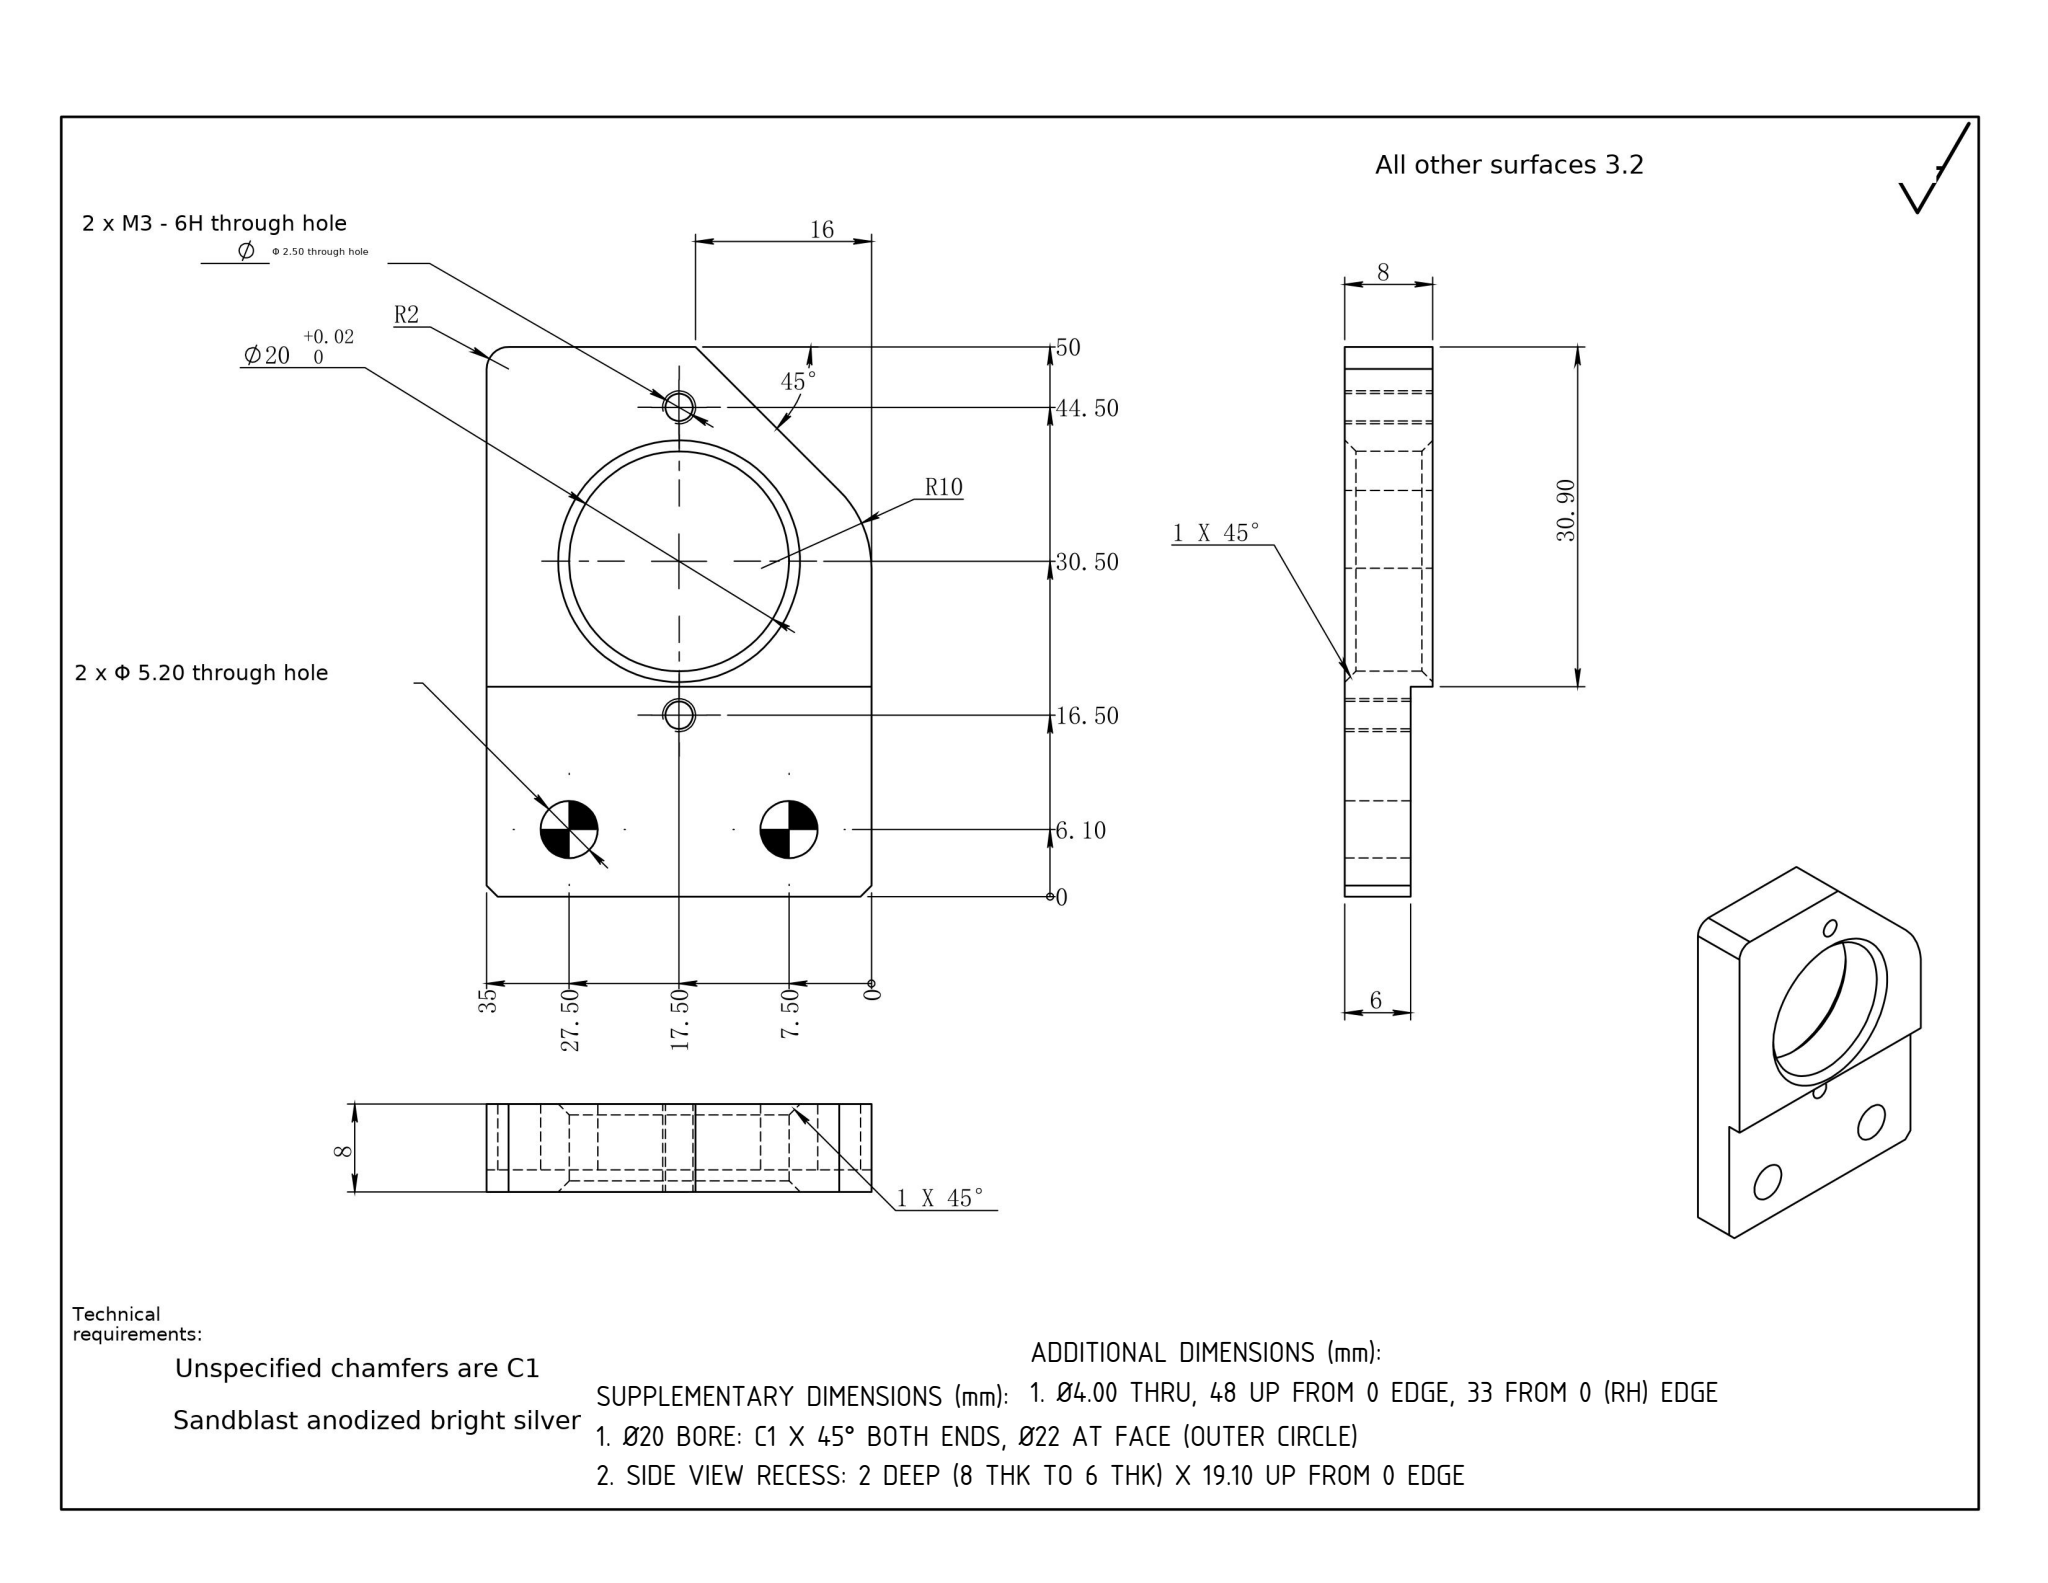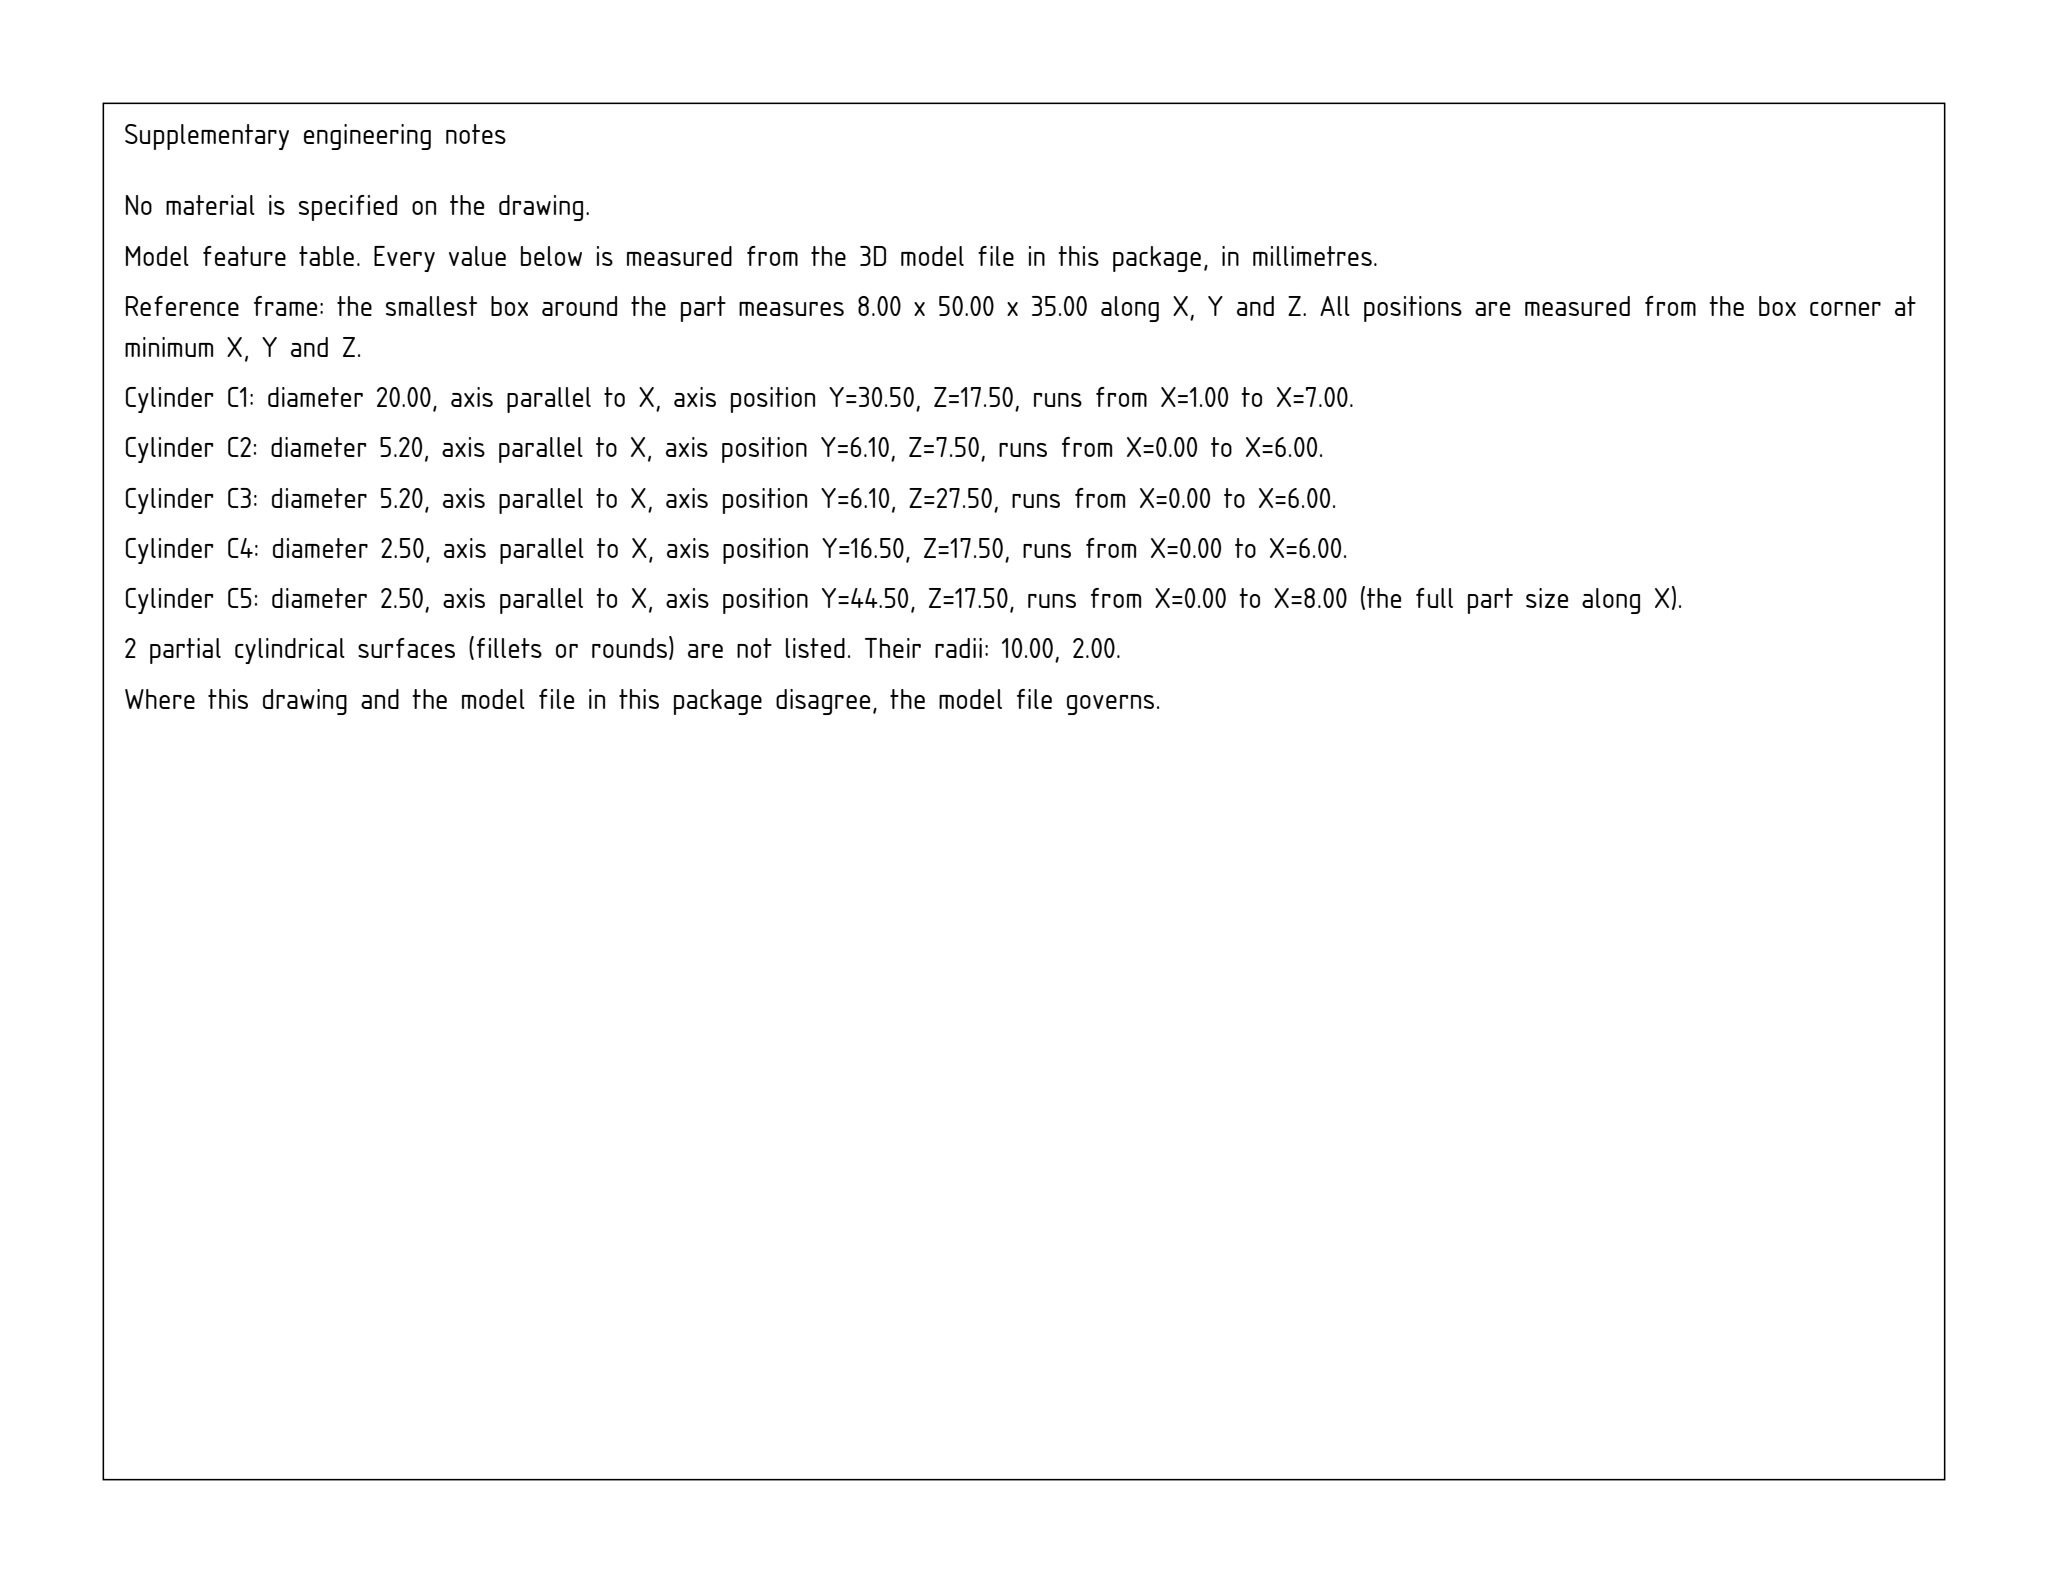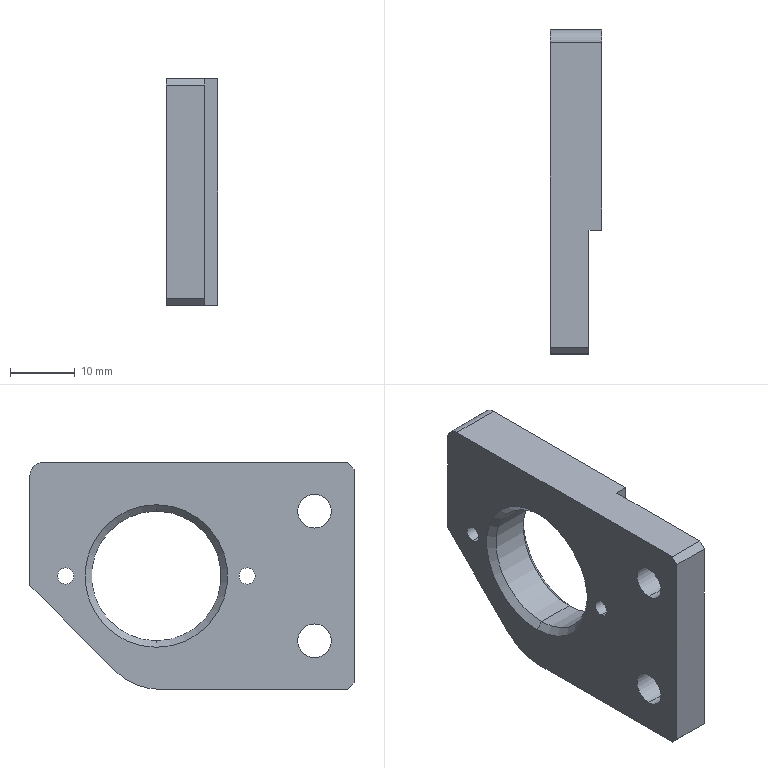Part | SolidWorks | mm | 1 solid | 27 faces | box 8 x 50 x 35 mm | volume 8707 mm3 | cylinder 12 | plane 11 | cone 4 | commonest cylinder face diameters 2.5 x4 5.2 x4 20 x3 4 x1
build123d program:
from build123d import *

# Parameters (mm, degrees)
SKETCH1_W                  = 35
SKETCH1_H                  = 50
BOSS_EXTRUDE1_DEPTH        = 4
SKETCH2_W                  = 2
SKETCH2_H                  = 19.1
CUT_EXTRUDE1_DEPTH         = 44.197
CHAMFER1_SIZE              = 1
SKETCH3_R                  = 10
CUT_EXTRUDE2_DEPTH         = 32.548
F_5_2_5_2_DIAMETER_HOLE1_D = 5.2
M3_TAPPED_HOLE1_D          = 2.5
CHAMFER2_SIZE              = 1
CHAMFER3_SIZE              = 16
FILLET1_R                  = 10
FILLET2_R                  = 2


with BuildPart() as part:
    # Sketch1 → Boss-Extrude1 (new, symmetric)
    with BuildSketch(Plane(origin=(0, 0, 0), x_dir=(0, 0, -1), z_dir=(1, 0, 0))):
        Rectangle(SKETCH1_W, SKETCH1_H)
    extrude(amount=BOSS_EXTRUDE1_DEPTH, both=True)

    # Sketch2 → Cut-Extrude1 (cut, through all)
    with BuildSketch(Plane.XY.offset(17.5)):
        with Locations((3, -15.45)):
            Rectangle(SKETCH2_W, SKETCH2_H)
    extrude(amount=-CUT_EXTRUDE1_DEPTH, mode=Mode.SUBTRACT)

    # Chamfer1
    chamfer1_edges = [part.edges().sort_by_distance(p)[0] for p in [
        (-1, -25, -17.5),
        (-1, -25, 17.5),
    ]]
    chamfer(chamfer1_edges, length=CHAMFER1_SIZE)

    # Sketch3 → Cut-Extrude2 (cut, through all)
    with BuildSketch(Plane.ZY.offset(4)):
        with Locations((0, 5.5)):
            Circle(SKETCH3_R)
    extrude(amount=-CUT_EXTRUDE2_DEPTH, mode=Mode.SUBTRACT)

    # 5.2 _5.2_ Diameter Hole1 (through all)
    with Locations(Plane.ZY.offset(4)):
        with Locations((-10, -18.9), (10, -18.9)):
            Hole(F_5_2_5_2_DIAMETER_HOLE1_D / 2)

    # M3 Tapped Hole1 (through all)
    with Locations(Plane.ZY.offset(4)):
        with Locations((0, -8.5), (0, 19.5)):
            Hole(M3_TAPPED_HOLE1_D / 2)

    # Chamfer2
    chamfer2_edges = [part.edges().sort_by_distance(p)[0] for p in [
        (4, 5.5, -10),
        (-4, 5.5, -10),
    ]]
    chamfer(chamfer2_edges, length=CHAMFER2_SIZE)

    # Chamfer3
    chamfer3_edges = [part.edges().sort_by_distance(p)[0] for p in [
        (0, 25, -17.5),
    ]]
    chamfer(chamfer3_edges, length=CHAMFER3_SIZE)

    # Fillet1
    fillet1_edges = [part.edges().sort_by_distance(p)[0] for p in [
        (0, 9, -17.5),
    ]]
    fillet(fillet1_edges, radius=FILLET1_R)

    # Fillet2
    fillet2_edges = [part.edges().sort_by_distance(p)[0] for p in [
        (0, 25, 17.5),
    ]]
    fillet(fillet2_edges, radius=FILLET2_R)


solid = part.part
STEP:
#1=CARTESIAN_POINT('',(3.,5.5,10.));
#2=VERTEX_POINT('',#1);
#3=CARTESIAN_POINT('',(3.,5.5,-10.));
#4=VERTEX_POINT('',#3);
#5=CARTESIAN_POINT('',(3.,5.5,0.));
#6=DIRECTION('',(1.,0.,0.));
#7=DIRECTION('',(0.,0.,1.));
#8=AXIS2_PLACEMENT_3D('',#5,#6,#7);
#9=CIRCLE('',#8,10.);
#10=EDGE_CURVE('',#2,#4,#9,.T.);
#11=ORIENTED_EDGE('',*,*,#10,.F.);
#12=CARTESIAN_POINT('',(4.,5.5,11.));
#13=VERTEX_POINT('',#12);
#14=CARTESIAN_POINT('',(4.,5.5,11.));
#15=DIRECTION('',(0.7071,0.,0.7071));
#16=VECTOR('',#15,1000.);
#17=LINE('',#14,#16);
#18=EDGE_CURVE('',#2,#13,#17,.T.);
#19=ORIENTED_EDGE('',*,*,#18,.T.);
#20=CARTESIAN_POINT('',(4.,5.5,-11.));
#21=VERTEX_POINT('',#20);
#22=CARTESIAN_POINT('',(4.,5.5,0.));
#23=DIRECTION('',(-1.,0.,0.));
#24=DIRECTION('',(0.,0.,1.));
#25=AXIS2_PLACEMENT_3D('',#22,#23,#24);
#26=CIRCLE('',#25,11.);
#27=EDGE_CURVE('',#21,#13,#26,.T.);
#28=ORIENTED_EDGE('',*,*,#27,.F.);
#29=CARTESIAN_POINT('',(4.,5.5,-11.));
#30=DIRECTION('',(0.7071,0.,-0.7071));
#31=VECTOR('',#30,1000.);
#32=LINE('',#29,#31);
#33=EDGE_CURVE('',#4,#21,#32,.T.);
#34=ORIENTED_EDGE('',*,*,#33,.F.);
#35=EDGE_LOOP('',(#11,#19,#28,#34));
#36=FACE_OUTER_BOUND('',#35,.T.);
#37=CARTESIAN_POINT('',(4.,5.5,0.));
#38=DIRECTION('',(1.,0.,0.));
#39=DIRECTION('',(0.,0.,-1.));
#40=AXIS2_PLACEMENT_3D('',#37,#38,#39);
#41=CONICAL_SURFACE('',#40,11.,0.7854);
#42=ADVANCED_FACE('',(#36),#41,.F.);
#43=CARTESIAN_POINT('',(-3.,5.5,-10.));
#44=VERTEX_POINT('',#43);
#45=CARTESIAN_POINT('',(-3.,5.5,10.));
#46=VERTEX_POINT('',#45);
#47=CARTESIAN_POINT('',(-3.,5.5,0.));
#48=DIRECTION('',(-1.,0.,0.));
#49=DIRECTION('',(0.,0.,1.));
#50=AXIS2_PLACEMENT_3D('',#47,#48,#49);
#51=CIRCLE('',#50,10.);
#52=EDGE_CURVE('',#44,#46,#51,.T.);
#53=ORIENTED_EDGE('',*,*,#52,.F.);
#54=CARTESIAN_POINT('',(-4.,5.5,-11.));
#55=VERTEX_POINT('',#54);
#56=CARTESIAN_POINT('',(-3.,5.5,-10.));
#57=DIRECTION('',(-0.7071,0.,-0.7071));
#58=VECTOR('',#57,1000.);
#59=LINE('',#56,#58);
#60=EDGE_CURVE('',#44,#55,#59,.T.);
#61=ORIENTED_EDGE('',*,*,#60,.T.);
#62=CARTESIAN_POINT('',(-4.,5.5,11.));
#63=VERTEX_POINT('',#62);
#64=CARTESIAN_POINT('',(-4.,5.5,0.));
#65=DIRECTION('',(1.,0.,0.));
#66=DIRECTION('',(0.,0.,1.));
#67=AXIS2_PLACEMENT_3D('',#64,#65,#66);
#68=CIRCLE('',#67,11.);
#69=EDGE_CURVE('',#63,#55,#68,.T.);
#70=ORIENTED_EDGE('',*,*,#69,.F.);
#71=CARTESIAN_POINT('',(-3.,5.5,10.));
#72=DIRECTION('',(-0.7071,0.,0.7071));
#73=VECTOR('',#72,1000.);
#74=LINE('',#71,#73);
#75=EDGE_CURVE('',#46,#63,#74,.T.);
#76=ORIENTED_EDGE('',*,*,#75,.F.);
#77=EDGE_LOOP('',(#53,#61,#70,#76));
#78=FACE_OUTER_BOUND('',#77,.T.);
#79=CARTESIAN_POINT('',(-3.,5.5,0.));
#80=DIRECTION('',(-1.,0.,0.));
#81=DIRECTION('',(0.,0.,1.));
#82=AXIS2_PLACEMENT_3D('',#79,#80,#81);
#83=CONICAL_SURFACE('',#82,10.,0.7854);
#84=ADVANCED_FACE('',(#78),#83,.F.);
#85=CARTESIAN_POINT('',(2.,-8.5,-1.25));
#86=VERTEX_POINT('',#85);
#87=CARTESIAN_POINT('',(2.,-8.5,1.25));
#88=VERTEX_POINT('',#87);
#89=CARTESIAN_POINT('',(2.,-8.5,0.));
#90=DIRECTION('',(-1.,0.,0.));
#91=DIRECTION('',(0.,0.,1.));
#92=AXIS2_PLACEMENT_3D('',#89,#90,#91);
#93=CIRCLE('',#92,1.25);
#94=EDGE_CURVE('',#86,#88,#93,.T.);
#95=ORIENTED_EDGE('',*,*,#94,.F.);
#96=CARTESIAN_POINT('',(-4.,-8.5,-1.25));
#97=VERTEX_POINT('',#96);
#98=CARTESIAN_POINT('',(-4.,-8.5,-1.25));
#99=DIRECTION('',(-1.,0.,0.));
#100=VECTOR('',#99,1000.);
#101=LINE('',#98,#100);
#102=EDGE_CURVE('',#86,#97,#101,.T.);
#103=ORIENTED_EDGE('',*,*,#102,.T.);
#104=CARTESIAN_POINT('',(-4.,-8.5,1.25));
#105=VERTEX_POINT('',#104);
#106=CARTESIAN_POINT('',(-4.,-8.5,0.));
#107=DIRECTION('',(-1.,0.,0.));
#108=DIRECTION('',(0.,0.,1.));
#109=AXIS2_PLACEMENT_3D('',#106,#107,#108);
#110=CIRCLE('',#109,1.25);
#111=EDGE_CURVE('',#97,#105,#110,.T.);
#112=ORIENTED_EDGE('',*,*,#111,.T.);
#113=CARTESIAN_POINT('',(-4.,-8.5,1.25));
#114=DIRECTION('',(-1.,0.,0.));
#115=VECTOR('',#114,1000.);
#116=LINE('',#113,#115);
#117=EDGE_CURVE('',#88,#105,#116,.T.);
#118=ORIENTED_EDGE('',*,*,#117,.F.);
#119=EDGE_LOOP('',(#95,#103,#112,#118));
#120=FACE_OUTER_BOUND('',#119,.T.);
#121=CARTESIAN_POINT('',(-4.,-8.5,0.));
#122=DIRECTION('',(-1.,0.,0.));
#123=DIRECTION('',(0.,0.,1.));
#124=AXIS2_PLACEMENT_3D('',#121,#122,#123);
#125=CYLINDRICAL_SURFACE('',#124,1.25);
#126=ADVANCED_FACE('',(#120),#125,.F.);
#127=CARTESIAN_POINT('',(4.,19.5,-1.25));
#128=VERTEX_POINT('',#127);
#129=CARTESIAN_POINT('',(4.,19.5,1.25));
#130=VERTEX_POINT('',#129);
#131=CARTESIAN_POINT('',(4.,19.5,-0.));
#132=DIRECTION('',(-1.,0.,0.));
#133=DIRECTION('',(0.,0.,1.));
#134=AXIS2_PLACEMENT_3D('',#131,#132,#133);
#135=CIRCLE('',#134,1.25);
#136=EDGE_CURVE('',#128,#130,#135,.T.);
#137=ORIENTED_EDGE('',*,*,#136,.F.);
#138=CARTESIAN_POINT('',(-4.,19.5,-1.25));
#139=VERTEX_POINT('',#138);
#140=CARTESIAN_POINT('',(-4.,19.5,-1.25));
#141=DIRECTION('',(-1.,0.,0.));
#142=VECTOR('',#141,1000.);
#143=LINE('',#140,#142);
#144=EDGE_CURVE('',#128,#139,#143,.T.);
#145=ORIENTED_EDGE('',*,*,#144,.T.);
#146=CARTESIAN_POINT('',(-4.,19.5,1.25));
#147=VERTEX_POINT('',#146);
#148=CARTESIAN_POINT('',(-4.,19.5,-0.));
#149=DIRECTION('',(-1.,0.,0.));
#150=DIRECTION('',(0.,0.,1.));
#151=AXIS2_PLACEMENT_3D('',#148,#149,#150);
#152=CIRCLE('',#151,1.25);
#153=EDGE_CURVE('',#139,#147,#152,.T.);
#154=ORIENTED_EDGE('',*,*,#153,.T.);
#155=CARTESIAN_POINT('',(-4.,19.5,1.25));
#156=DIRECTION('',(-1.,0.,0.));
#157=VECTOR('',#156,1000.);
#158=LINE('',#155,#157);
#159=EDGE_CURVE('',#130,#147,#158,.T.);
#160=ORIENTED_EDGE('',*,*,#159,.F.);
#161=EDGE_LOOP('',(#137,#145,#154,#160));
#162=FACE_OUTER_BOUND('',#161,.T.);
#163=CARTESIAN_POINT('',(-4.,19.5,-0.));
#164=DIRECTION('',(-1.,0.,0.));
#165=DIRECTION('',(0.,0.,1.));
#166=AXIS2_PLACEMENT_3D('',#163,#164,#165);
#167=CYLINDRICAL_SURFACE('',#166,1.25);
#168=ADVANCED_FACE('',(#162),#167,.F.);
#169=CARTESIAN_POINT('',(2.,-18.9,-12.6));
#170=VERTEX_POINT('',#169);
#171=CARTESIAN_POINT('',(2.,-18.9,-7.4));
#172=VERTEX_POINT('',#171);
#173=CARTESIAN_POINT('',(2.,-18.9,-10.));
#174=DIRECTION('',(-1.,0.,0.));
#175=DIRECTION('',(0.,0.,1.));
#176=AXIS2_PLACEMENT_3D('',#173,#174,#175);
#177=CIRCLE('',#176,2.6);
#178=EDGE_CURVE('',#170,#172,#177,.T.);
#179=ORIENTED_EDGE('',*,*,#178,.F.);
#180=CARTESIAN_POINT('',(-4.,-18.9,-12.6));
#181=VERTEX_POINT('',#180);
#182=CARTESIAN_POINT('',(-4.,-18.9,-12.6));
#183=DIRECTION('',(-1.,0.,0.));
#184=VECTOR('',#183,1000.);
#185=LINE('',#182,#184);
#186=EDGE_CURVE('',#170,#181,#185,.T.);
#187=ORIENTED_EDGE('',*,*,#186,.T.);
#188=CARTESIAN_POINT('',(-4.,-18.9,-7.4));
#189=VERTEX_POINT('',#188);
#190=CARTESIAN_POINT('',(-4.,-18.9,-10.));
#191=DIRECTION('',(-1.,0.,0.));
#192=DIRECTION('',(0.,0.,1.));
#193=AXIS2_PLACEMENT_3D('',#190,#191,#192);
#194=CIRCLE('',#193,2.6);
#195=EDGE_CURVE('',#181,#189,#194,.T.);
#196=ORIENTED_EDGE('',*,*,#195,.T.);
#197=CARTESIAN_POINT('',(-4.,-18.9,-7.4));
#198=DIRECTION('',(-1.,0.,0.));
#199=VECTOR('',#198,1000.);
#200=LINE('',#197,#199);
#201=EDGE_CURVE('',#172,#189,#200,.T.);
#202=ORIENTED_EDGE('',*,*,#201,.F.);
#203=EDGE_LOOP('',(#179,#187,#196,#202));
#204=FACE_OUTER_BOUND('',#203,.T.);
#205=CARTESIAN_POINT('',(-4.,-18.9,-10.));
#206=DIRECTION('',(-1.,0.,0.));
#207=DIRECTION('',(0.,0.,1.));
#208=AXIS2_PLACEMENT_3D('',#205,#206,#207);
#209=CYLINDRICAL_SURFACE('',#208,2.6);
#210=ADVANCED_FACE('',(#204),#209,.F.);
#211=CARTESIAN_POINT('',(2.,-18.9,7.4));
#212=VERTEX_POINT('',#211);
#213=CARTESIAN_POINT('',(2.,-18.9,12.6));
#214=VERTEX_POINT('',#213);
#215=CARTESIAN_POINT('',(2.,-18.9,10.));
#216=DIRECTION('',(-1.,0.,0.));
#217=DIRECTION('',(0.,0.,1.));
#218=AXIS2_PLACEMENT_3D('',#215,#216,#217);
#219=CIRCLE('',#218,2.6);
#220=EDGE_CURVE('',#212,#214,#219,.T.);
#221=ORIENTED_EDGE('',*,*,#220,.F.);
#222=CARTESIAN_POINT('',(-4.,-18.9,7.4));
#223=VERTEX_POINT('',#222);
#224=CARTESIAN_POINT('',(-4.,-18.9,7.4));
#225=DIRECTION('',(-1.,0.,0.));
#226=VECTOR('',#225,1000.);
#227=LINE('',#224,#226);
#228=EDGE_CURVE('',#212,#223,#227,.T.);
#229=ORIENTED_EDGE('',*,*,#228,.T.);
#230=CARTESIAN_POINT('',(-4.,-18.9,12.6));
#231=VERTEX_POINT('',#230);
#232=CARTESIAN_POINT('',(-4.,-18.9,10.));
#233=DIRECTION('',(-1.,0.,0.));
#234=DIRECTION('',(0.,0.,1.));
#235=AXIS2_PLACEMENT_3D('',#232,#233,#234);
#236=CIRCLE('',#235,2.6);
#237=EDGE_CURVE('',#223,#231,#236,.T.);
#238=ORIENTED_EDGE('',*,*,#237,.T.);
#239=CARTESIAN_POINT('',(-4.,-18.9,12.6));
#240=DIRECTION('',(-1.,0.,0.));
#241=VECTOR('',#240,1000.);
#242=LINE('',#239,#241);
#243=EDGE_CURVE('',#214,#231,#242,.T.);
#244=ORIENTED_EDGE('',*,*,#243,.F.);
#245=EDGE_LOOP('',(#221,#229,#238,#244));
#246=FACE_OUTER_BOUND('',#245,.T.);
#247=CARTESIAN_POINT('',(-4.,-18.9,10.));
#248=DIRECTION('',(-1.,0.,0.));
#249=DIRECTION('',(0.,0.,1.));
#250=AXIS2_PLACEMENT_3D('',#247,#248,#249);
#251=CYLINDRICAL_SURFACE('',#250,2.6);
#252=ADVANCED_FACE('',(#246),#251,.F.);
#253=ORIENTED_EDGE('',*,*,#10,.T.);
#254=CARTESIAN_POINT('',(4.,5.5,-10.));
#255=DIRECTION('',(-1.,0.,0.));
#256=VECTOR('',#255,1000.);
#257=LINE('',#254,#256);
#258=EDGE_CURVE('',#4,#44,#257,.T.);
#259=ORIENTED_EDGE('',*,*,#258,.T.);
#260=ORIENTED_EDGE('',*,*,#52,.T.);
#261=CARTESIAN_POINT('',(4.,5.5,10.));
#262=DIRECTION('',(-1.,0.,0.));
#263=VECTOR('',#262,1000.);
#264=LINE('',#261,#263);
#265=EDGE_CURVE('',#2,#46,#264,.T.);
#266=ORIENTED_EDGE('',*,*,#265,.F.);
#267=EDGE_LOOP('',(#253,#259,#260,#266));
#268=FACE_OUTER_BOUND('',#267,.T.);
#269=CARTESIAN_POINT('',(4.,5.5,0.));
#270=DIRECTION('',(-1.,0.,0.));
#271=DIRECTION('',(0.,0.,1.));
#272=AXIS2_PLACEMENT_3D('',#269,#270,#271);
#273=CYLINDRICAL_SURFACE('',#272,10.);
#274=ADVANCED_FACE('',(#268),#273,.F.);
#275=CARTESIAN_POINT('',(-4.,-24.,-17.5));
#276=VERTEX_POINT('',#275);
#277=CARTESIAN_POINT('',(-4.,4.858,-17.5));
#278=VERTEX_POINT('',#277);
#279=CARTESIAN_POINT('',(-4.,-25.,-17.5));
#280=DIRECTION('',(0.,1.,0.));
#281=VECTOR('',#280,1000.);
#282=LINE('',#279,#281);
#283=EDGE_CURVE('',#276,#278,#282,.T.);
#284=ORIENTED_EDGE('',*,*,#283,.T.);
#285=CARTESIAN_POINT('',(4.,4.858,-17.5));
#286=VERTEX_POINT('',#285);
#287=CARTESIAN_POINT('',(-4.,4.858,-17.5));
#288=DIRECTION('',(1.,0.,0.));
#289=VECTOR('',#288,1000.);
#290=LINE('',#287,#289);
#291=EDGE_CURVE('',#278,#286,#290,.T.);
#292=ORIENTED_EDGE('',*,*,#291,.T.);
#293=CARTESIAN_POINT('',(4.,-5.9,-17.5));
#294=VERTEX_POINT('',#293);
#295=CARTESIAN_POINT('',(4.,-25.,-17.5));
#296=DIRECTION('',(0.,1.,0.));
#297=VECTOR('',#296,1000.);
#298=LINE('',#295,#297);
#299=EDGE_CURVE('',#294,#286,#298,.T.);
#300=ORIENTED_EDGE('',*,*,#299,.F.);
#301=CARTESIAN_POINT('',(2.,-5.9,-17.5));
#302=VERTEX_POINT('',#301);
#303=CARTESIAN_POINT('',(4.,-5.9,-17.5));
#304=DIRECTION('',(-1.,0.,0.));
#305=VECTOR('',#304,1000.);
#306=LINE('',#303,#305);
#307=EDGE_CURVE('',#294,#302,#306,.T.);
#308=ORIENTED_EDGE('',*,*,#307,.T.);
#309=CARTESIAN_POINT('',(2.,-24.,-17.5));
#310=VERTEX_POINT('',#309);
#311=CARTESIAN_POINT('',(2.,-25.,-17.5));
#312=DIRECTION('',(0.,-1.,0.));
#313=VECTOR('',#312,1000.);
#314=LINE('',#311,#313);
#315=EDGE_CURVE('',#302,#310,#314,.T.);
#316=ORIENTED_EDGE('',*,*,#315,.T.);
#317=CARTESIAN_POINT('',(-4.,-24.,-17.5));
#318=DIRECTION('',(-1.,0.,0.));
#319=VECTOR('',#318,1000.);
#320=LINE('',#317,#319);
#321=EDGE_CURVE('',#310,#276,#320,.T.);
#322=ORIENTED_EDGE('',*,*,#321,.T.);
#323=EDGE_LOOP('',(#284,#292,#300,#308,#316,#322));
#324=FACE_OUTER_BOUND('',#323,.T.);
#325=CARTESIAN_POINT('',(-4.,-25.,-17.5));
#326=DIRECTION('',(0.,0.,-1.));
#327=DIRECTION('',(-1.,0.,0.));
#328=AXIS2_PLACEMENT_3D('',#325,#326,#327);
#329=PLANE('',#328);
#330=ADVANCED_FACE('',(#324),#329,.T.);
#331=CARTESIAN_POINT('',(-4.,-25.,16.5));
#332=VERTEX_POINT('',#331);
#333=CARTESIAN_POINT('',(-4.,-25.,-16.5));
#334=VERTEX_POINT('',#333);
#335=CARTESIAN_POINT('',(-4.,-25.,17.5));
#336=DIRECTION('',(0.,0.,-1.));
#337=VECTOR('',#336,1000.);
#338=LINE('',#335,#337);
#339=EDGE_CURVE('',#332,#334,#338,.T.);
#340=ORIENTED_EDGE('',*,*,#339,.T.);
#341=CARTESIAN_POINT('',(2.,-25.,-16.5));
#342=VERTEX_POINT('',#341);
#343=CARTESIAN_POINT('',(-4.,-25.,-16.5));
#344=DIRECTION('',(1.,0.,0.));
#345=VECTOR('',#344,1000.);
#346=LINE('',#343,#345);
#347=EDGE_CURVE('',#334,#342,#346,.T.);
#348=ORIENTED_EDGE('',*,*,#347,.T.);
#349=CARTESIAN_POINT('',(2.,-25.,16.5));
#350=VERTEX_POINT('',#349);
#351=CARTESIAN_POINT('',(2.,-25.,-17.5));
#352=DIRECTION('',(0.,0.,1.));
#353=VECTOR('',#352,1000.);
#354=LINE('',#351,#353);
#355=EDGE_CURVE('',#342,#350,#354,.T.);
#356=ORIENTED_EDGE('',*,*,#355,.T.);
#357=CARTESIAN_POINT('',(-4.,-25.,16.5));
#358=DIRECTION('',(-1.,0.,0.));
#359=VECTOR('',#358,1000.);
#360=LINE('',#357,#359);
#361=EDGE_CURVE('',#350,#332,#360,.T.);
#362=ORIENTED_EDGE('',*,*,#361,.T.);
#363=EDGE_LOOP('',(#340,#348,#356,#362));
#364=FACE_OUTER_BOUND('',#363,.T.);
#365=CARTESIAN_POINT('',(-4.,-25.,17.5));
#366=DIRECTION('',(0.,-1.,0.));
#367=DIRECTION('',(0.,0.,-1.));
#368=AXIS2_PLACEMENT_3D('',#365,#366,#367);
#369=PLANE('',#368);
#370=ADVANCED_FACE('',(#364),#369,.T.);
#371=CARTESIAN_POINT('',(4.,23.,17.5));
#372=VERTEX_POINT('',#371);
#373=CARTESIAN_POINT('',(4.,-5.9,17.5));
#374=VERTEX_POINT('',#373);
#375=CARTESIAN_POINT('',(4.,-25.,17.5));
#376=DIRECTION('',(0.,-1.,0.));
#377=VECTOR('',#376,1000.);
#378=LINE('',#375,#377);
#379=EDGE_CURVE('',#372,#374,#378,.T.);
#380=ORIENTED_EDGE('',*,*,#379,.F.);
#381=CARTESIAN_POINT('',(-4.,23.,17.5));
#382=VERTEX_POINT('',#381);
#383=CARTESIAN_POINT('',(-4.,23.,17.5));
#384=DIRECTION('',(-1.,0.,0.));
#385=VECTOR('',#384,1000.);
#386=LINE('',#383,#385);
#387=EDGE_CURVE('',#372,#382,#386,.T.);
#388=ORIENTED_EDGE('',*,*,#387,.T.);
#389=CARTESIAN_POINT('',(-4.,-24.,17.5));
#390=VERTEX_POINT('',#389);
#391=CARTESIAN_POINT('',(-4.,-25.,17.5));
#392=DIRECTION('',(0.,-1.,0.));
#393=VECTOR('',#392,1000.);
#394=LINE('',#391,#393);
#395=EDGE_CURVE('',#382,#390,#394,.T.);
#396=ORIENTED_EDGE('',*,*,#395,.T.);
#397=CARTESIAN_POINT('',(2.,-24.,17.5));
#398=VERTEX_POINT('',#397);
#399=CARTESIAN_POINT('',(-4.,-24.,17.5));
#400=DIRECTION('',(1.,0.,0.));
#401=VECTOR('',#400,1000.);
#402=LINE('',#399,#401);
#403=EDGE_CURVE('',#390,#398,#402,.T.);
#404=ORIENTED_EDGE('',*,*,#403,.T.);
#405=CARTESIAN_POINT('',(2.,-5.9,17.5));
#406=VERTEX_POINT('',#405);
#407=CARTESIAN_POINT('',(2.,-25.,17.5));
#408=DIRECTION('',(0.,-1.,0.));
#409=VECTOR('',#408,1000.);
#410=LINE('',#407,#409);
#411=EDGE_CURVE('',#406,#398,#410,.T.);
#412=ORIENTED_EDGE('',*,*,#411,.F.);
#413=CARTESIAN_POINT('',(4.,-5.9,17.5));
#414=DIRECTION('',(-1.,0.,0.));
#415=VECTOR('',#414,1000.);
#416=LINE('',#413,#415);
#417=EDGE_CURVE('',#374,#406,#416,.T.);
#418=ORIENTED_EDGE('',*,*,#417,.F.);
#419=EDGE_LOOP('',(#380,#388,#396,#404,#412,#418));
#420=FACE_OUTER_BOUND('',#419,.T.);
#421=CARTESIAN_POINT('',(-4.,-25.,17.5));
#422=DIRECTION('',(0.,0.,1.));
#423=DIRECTION('',(1.,0.,0.));
#424=AXIS2_PLACEMENT_3D('',#421,#422,#423);
#425=PLANE('',#424);
#426=ADVANCED_FACE('',(#420),#425,.T.);
#427=CARTESIAN_POINT('',(-4.,25.,-1.5));
#428=VERTEX_POINT('',#427);
#429=CARTESIAN_POINT('',(-4.,25.,15.5));
#430=VERTEX_POINT('',#429);
#431=CARTESIAN_POINT('',(-4.,25.,17.5));
#432=DIRECTION('',(0.,0.,1.));
#433=VECTOR('',#432,1000.);
#434=LINE('',#431,#433);
#435=EDGE_CURVE('',#428,#430,#434,.T.);
#436=ORIENTED_EDGE('',*,*,#435,.T.);
#437=CARTESIAN_POINT('',(4.,25.,15.5));
#438=VERTEX_POINT('',#437);
#439=CARTESIAN_POINT('',(-4.,25.,15.5));
#440=DIRECTION('',(1.,0.,0.));
#441=VECTOR('',#440,1000.);
#442=LINE('',#439,#441);
#443=EDGE_CURVE('',#430,#438,#442,.T.);
#444=ORIENTED_EDGE('',*,*,#443,.T.);
#445=CARTESIAN_POINT('',(4.,25.,-1.5));
#446=VERTEX_POINT('',#445);
#447=CARTESIAN_POINT('',(4.,25.,17.5));
#448=DIRECTION('',(0.,0.,1.));
#449=VECTOR('',#448,1000.);
#450=LINE('',#447,#449);
#451=EDGE_CURVE('',#446,#438,#450,.T.);
#452=ORIENTED_EDGE('',*,*,#451,.F.);
#453=CARTESIAN_POINT('',(-4.,25.,-1.5));
#454=DIRECTION('',(-1.,0.,0.));
#455=VECTOR('',#454,1000.);
#456=LINE('',#453,#455);
#457=EDGE_CURVE('',#446,#428,#456,.T.);
#458=ORIENTED_EDGE('',*,*,#457,.T.);
#459=EDGE_LOOP('',(#436,#444,#452,#458));
#460=FACE_OUTER_BOUND('',#459,.T.);
#461=CARTESIAN_POINT('',(-4.,25.,17.5));
#462=DIRECTION('',(0.,1.,0.));
#463=DIRECTION('',(0.,0.,1.));
#464=AXIS2_PLACEMENT_3D('',#461,#462,#463);
#465=PLANE('',#464);
#466=ADVANCED_FACE('',(#460),#465,.T.);
#467=ORIENTED_EDGE('',*,*,#69,.T.);
#468=CARTESIAN_POINT('',(-4.,5.5,0.));
#469=DIRECTION('',(1.,0.,0.));
#470=DIRECTION('',(0.,0.,1.));
#471=AXIS2_PLACEMENT_3D('',#468,#469,#470);
#472=CIRCLE('',#471,11.);
#473=EDGE_CURVE('',#55,#63,#472,.T.);
#474=ORIENTED_EDGE('',*,*,#473,.T.);
#475=EDGE_LOOP('',(#467,#474));
#476=FACE_BOUND('',#475,.T.);
#477=CARTESIAN_POINT('',(-4.,-8.5,0.));
#478=DIRECTION('',(-1.,0.,0.));
#479=DIRECTION('',(0.,0.,1.));
#480=AXIS2_PLACEMENT_3D('',#477,#478,#479);
#481=CIRCLE('',#480,1.25);
#482=EDGE_CURVE('',#105,#97,#481,.T.);
#483=ORIENTED_EDGE('',*,*,#482,.F.);
#484=ORIENTED_EDGE('',*,*,#111,.F.);
#485=EDGE_LOOP('',(#483,#484));
#486=FACE_BOUND('',#485,.T.);
#487=CARTESIAN_POINT('',(-4.,19.5,-0.));
#488=DIRECTION('',(-1.,0.,0.));
#489=DIRECTION('',(0.,0.,1.));
#490=AXIS2_PLACEMENT_3D('',#487,#488,#489);
#491=CIRCLE('',#490,1.25);
#492=EDGE_CURVE('',#147,#139,#491,.T.);
#493=ORIENTED_EDGE('',*,*,#492,.F.);
#494=ORIENTED_EDGE('',*,*,#153,.F.);
#495=EDGE_LOOP('',(#493,#494));
#496=FACE_BOUND('',#495,.T.);
#497=CARTESIAN_POINT('',(-4.,-18.9,-10.));
#498=DIRECTION('',(-1.,0.,0.));
#499=DIRECTION('',(0.,0.,1.));
#500=AXIS2_PLACEMENT_3D('',#497,#498,#499);
#501=CIRCLE('',#500,2.6);
#502=EDGE_CURVE('',#189,#181,#501,.T.);
#503=ORIENTED_EDGE('',*,*,#502,.F.);
#504=ORIENTED_EDGE('',*,*,#195,.F.);
#505=EDGE_LOOP('',(#503,#504));
#506=FACE_BOUND('',#505,.T.);
#507=CARTESIAN_POINT('',(-4.,-18.9,10.));
#508=DIRECTION('',(-1.,0.,0.));
#509=DIRECTION('',(0.,0.,1.));
#510=AXIS2_PLACEMENT_3D('',#507,#508,#509);
#511=CIRCLE('',#510,2.6);
#512=EDGE_CURVE('',#231,#223,#511,.T.);
#513=ORIENTED_EDGE('',*,*,#512,.F.);
#514=ORIENTED_EDGE('',*,*,#237,.F.);
#515=EDGE_LOOP('',(#513,#514));
#516=FACE_BOUND('',#515,.T.);
#517=ORIENTED_EDGE('',*,*,#395,.F.);
#518=CARTESIAN_POINT('',(-4.,23.,15.5));
#519=DIRECTION('',(-1.,0.,0.));
#520=DIRECTION('',(0.,0.,1.));
#521=AXIS2_PLACEMENT_3D('',#518,#519,#520);
#522=CIRCLE('',#521,2.);
#523=EDGE_CURVE('',#382,#430,#522,.T.);
#524=ORIENTED_EDGE('',*,*,#523,.T.);
#525=ORIENTED_EDGE('',*,*,#435,.F.);
#526=CARTESIAN_POINT('',(-4.,11.929,-14.571));
#527=VERTEX_POINT('',#526);
#528=CARTESIAN_POINT('',(-4.,13.25,-13.25));
#529=DIRECTION('',(0.,-0.7071,-0.7071));
#530=VECTOR('',#529,1000.);
#531=LINE('',#528,#530);
#532=EDGE_CURVE('',#428,#527,#531,.T.);
#533=ORIENTED_EDGE('',*,*,#532,.T.);
#534=CARTESIAN_POINT('',(-4.,4.858,-7.5));
#535=DIRECTION('',(-1.,0.,0.));
#536=DIRECTION('',(0.,0.,1.));
#537=AXIS2_PLACEMENT_3D('',#534,#535,#536);
#538=CIRCLE('',#537,10.);
#539=EDGE_CURVE('',#527,#278,#538,.T.);
#540=ORIENTED_EDGE('',*,*,#539,.T.);
#541=ORIENTED_EDGE('',*,*,#283,.F.);
#542=CARTESIAN_POINT('',(-4.,-20.75,-20.75));
#543=DIRECTION('',(0.,-0.7071,0.7071));
#544=VECTOR('',#543,1000.);
#545=LINE('',#542,#544);
#546=EDGE_CURVE('',#276,#334,#545,.T.);
#547=ORIENTED_EDGE('',*,*,#546,.T.);
#548=ORIENTED_EDGE('',*,*,#339,.F.);
#549=CARTESIAN_POINT('',(-4.,-20.75,20.75));
#550=DIRECTION('',(0.,0.7071,0.7071));
#551=VECTOR('',#550,1000.);
#552=LINE('',#549,#551);
#553=EDGE_CURVE('',#332,#390,#552,.T.);
#554=ORIENTED_EDGE('',*,*,#553,.T.);
#555=EDGE_LOOP('',(#517,#524,#525,#533,#540,#541,#547,#548,#554));
#556=FACE_OUTER_BOUND('',#555,.T.);
#557=CARTESIAN_POINT('',(-4.,0.,0.));
#558=DIRECTION('',(-1.,0.,0.));
#559=DIRECTION('',(0.,0.,1.));
#560=AXIS2_PLACEMENT_3D('',#557,#558,#559);
#561=PLANE('',#560);
#562=ADVANCED_FACE('',(#476,#486,#496,#506,#516,#556),#561,.T.);
#563=ORIENTED_EDGE('',*,*,#27,.T.);
#564=CARTESIAN_POINT('',(4.,5.5,0.));
#565=DIRECTION('',(-1.,0.,0.));
#566=DIRECTION('',(0.,0.,1.));
#567=AXIS2_PLACEMENT_3D('',#564,#565,#566);
#568=CIRCLE('',#567,11.);
#569=EDGE_CURVE('',#13,#21,#568,.T.);
#570=ORIENTED_EDGE('',*,*,#569,.T.);
#571=EDGE_LOOP('',(#563,#570));
#572=FACE_BOUND('',#571,.T.);
#573=CARTESIAN_POINT('',(4.,19.5,-0.));
#574=DIRECTION('',(-1.,0.,0.));
#575=DIRECTION('',(0.,0.,1.));
#576=AXIS2_PLACEMENT_3D('',#573,#574,#575);
#577=CIRCLE('',#576,1.25);
#578=EDGE_CURVE('',#130,#128,#577,.T.);
#579=ORIENTED_EDGE('',*,*,#578,.T.);
#580=ORIENTED_EDGE('',*,*,#136,.T.);
#581=EDGE_LOOP('',(#579,#580));
#582=FACE_BOUND('',#581,.T.);
#583=ORIENTED_EDGE('',*,*,#451,.T.);
#584=CARTESIAN_POINT('',(4.,23.,15.5));
#585=DIRECTION('',(1.,0.,0.));
#586=DIRECTION('',(0.,0.,1.));
#587=AXIS2_PLACEMENT_3D('',#584,#585,#586);
#588=CIRCLE('',#587,2.);
#589=EDGE_CURVE('',#438,#372,#588,.T.);
#590=ORIENTED_EDGE('',*,*,#589,.T.);
#591=ORIENTED_EDGE('',*,*,#379,.T.);
#592=CARTESIAN_POINT('',(4.,-5.9,-17.5));
#593=DIRECTION('',(0.,0.,1.));
#594=VECTOR('',#593,1000.);
#595=LINE('',#592,#594);
#596=EDGE_CURVE('',#294,#374,#595,.T.);
#597=ORIENTED_EDGE('',*,*,#596,.F.);
#598=ORIENTED_EDGE('',*,*,#299,.T.);
#599=CARTESIAN_POINT('',(4.,11.929,-14.571));
#600=VERTEX_POINT('',#599);
#601=CARTESIAN_POINT('',(4.,4.858,-7.5));
#602=DIRECTION('',(1.,0.,0.));
#603=DIRECTION('',(0.,0.,1.));
#604=AXIS2_PLACEMENT_3D('',#601,#602,#603);
#605=CIRCLE('',#604,10.);
#606=EDGE_CURVE('',#286,#600,#605,.T.);
#607=ORIENTED_EDGE('',*,*,#606,.T.);
#608=CARTESIAN_POINT('',(4.,9.,-17.5));
#609=DIRECTION('',(0.,0.7071,0.7071));
#610=VECTOR('',#609,1000.);
#611=LINE('',#608,#610);
#612=EDGE_CURVE('',#600,#446,#611,.T.);
#613=ORIENTED_EDGE('',*,*,#612,.T.);
#614=EDGE_LOOP('',(#583,#590,#591,#597,#598,#607,#613));
#615=FACE_OUTER_BOUND('',#614,.T.);
#616=CARTESIAN_POINT('',(4.,0.,0.));
#617=DIRECTION('',(-1.,0.,0.));
#618=DIRECTION('',(0.,0.,1.));
#619=AXIS2_PLACEMENT_3D('',#616,#617,#618);
#620=PLANE('',#619);
#621=ADVANCED_FACE('',(#572,#582,#615),#620,.F.);
#622=CARTESIAN_POINT('',(2.,-8.5,0.));
#623=DIRECTION('',(-1.,0.,0.));
#624=DIRECTION('',(0.,0.,1.));
#625=AXIS2_PLACEMENT_3D('',#622,#623,#624);
#626=CIRCLE('',#625,1.25);
#627=EDGE_CURVE('',#88,#86,#626,.T.);
#628=ORIENTED_EDGE('',*,*,#627,.T.);
#629=ORIENTED_EDGE('',*,*,#94,.T.);
#630=EDGE_LOOP('',(#628,#629));
#631=FACE_BOUND('',#630,.T.);
#632=CARTESIAN_POINT('',(2.,-18.9,-10.));
#633=DIRECTION('',(-1.,0.,0.));
#634=DIRECTION('',(0.,0.,1.));
#635=AXIS2_PLACEMENT_3D('',#632,#633,#634);
#636=CIRCLE('',#635,2.6);
#637=EDGE_CURVE('',#172,#170,#636,.T.);
#638=ORIENTED_EDGE('',*,*,#637,.T.);
#639=ORIENTED_EDGE('',*,*,#178,.T.);
#640=EDGE_LOOP('',(#638,#639));
#641=FACE_BOUND('',#640,.T.);
#642=CARTESIAN_POINT('',(2.,-18.9,10.));
#643=DIRECTION('',(-1.,0.,0.));
#644=DIRECTION('',(0.,0.,1.));
#645=AXIS2_PLACEMENT_3D('',#642,#643,#644);
#646=CIRCLE('',#645,2.6);
#647=EDGE_CURVE('',#214,#212,#646,.T.);
#648=ORIENTED_EDGE('',*,*,#647,.T.);
#649=ORIENTED_EDGE('',*,*,#220,.T.);
#650=EDGE_LOOP('',(#648,#649));
#651=FACE_BOUND('',#650,.T.);
#652=ORIENTED_EDGE('',*,*,#355,.F.);
#653=CARTESIAN_POINT('',(2.,-25.,-16.5));
#654=DIRECTION('',(0.,0.7071,-0.7071));
#655=VECTOR('',#654,1000.);
#656=LINE('',#653,#655);
#657=EDGE_CURVE('',#342,#310,#656,.T.);
#658=ORIENTED_EDGE('',*,*,#657,.T.);
#659=ORIENTED_EDGE('',*,*,#315,.F.);
#660=CARTESIAN_POINT('',(2.,-5.9,-17.5));
#661=DIRECTION('',(0.,0.,1.));
#662=VECTOR('',#661,1000.);
#663=LINE('',#660,#662);
#664=EDGE_CURVE('',#302,#406,#663,.T.);
#665=ORIENTED_EDGE('',*,*,#664,.T.);
#666=ORIENTED_EDGE('',*,*,#411,.T.);
#667=CARTESIAN_POINT('',(2.,-24.,17.5));
#668=DIRECTION('',(0.,-0.7071,-0.7071));
#669=VECTOR('',#668,1000.);
#670=LINE('',#667,#669);
#671=EDGE_CURVE('',#398,#350,#670,.T.);
#672=ORIENTED_EDGE('',*,*,#671,.T.);
#673=EDGE_LOOP('',(#652,#658,#659,#665,#666,#672));
#674=FACE_OUTER_BOUND('',#673,.T.);
#675=CARTESIAN_POINT('',(2.,-25.,-17.5));
#676=DIRECTION('',(-1.,0.,0.));
#677=DIRECTION('',(0.,0.,1.));
#678=AXIS2_PLACEMENT_3D('',#675,#676,#677);
#679=PLANE('',#678);
#680=ADVANCED_FACE('',(#631,#641,#651,#674),#679,.F.);
#681=ORIENTED_EDGE('',*,*,#417,.T.);
#682=ORIENTED_EDGE('',*,*,#664,.F.);
#683=ORIENTED_EDGE('',*,*,#307,.F.);
#684=ORIENTED_EDGE('',*,*,#596,.T.);
#685=EDGE_LOOP('',(#681,#682,#683,#684));
#686=FACE_OUTER_BOUND('',#685,.T.);
#687=CARTESIAN_POINT('',(4.,-5.9,-17.5));
#688=DIRECTION('',(0.,1.,0.));
#689=DIRECTION('',(0.,0.,1.));
#690=AXIS2_PLACEMENT_3D('',#687,#688,#689);
#691=PLANE('',#690);
#692=ADVANCED_FACE('',(#686),#691,.F.);
#693=ORIENTED_EDGE('',*,*,#546,.F.);
#694=ORIENTED_EDGE('',*,*,#321,.F.);
#695=ORIENTED_EDGE('',*,*,#657,.F.);
#696=ORIENTED_EDGE('',*,*,#347,.F.);
#697=EDGE_LOOP('',(#693,#694,#695,#696));
#698=FACE_OUTER_BOUND('',#697,.T.);
#699=CARTESIAN_POINT('',(-4.,-25.,-16.5));
#700=DIRECTION('',(0.,0.7071,0.7071));
#701=DIRECTION('',(1.,0.,0.));
#702=AXIS2_PLACEMENT_3D('',#699,#700,#701);
#703=PLANE('',#702);
#704=ADVANCED_FACE('',(#698),#703,.F.);
#705=ORIENTED_EDGE('',*,*,#553,.F.);
#706=ORIENTED_EDGE('',*,*,#361,.F.);
#707=ORIENTED_EDGE('',*,*,#671,.F.);
#708=ORIENTED_EDGE('',*,*,#403,.F.);
#709=EDGE_LOOP('',(#705,#706,#707,#708));
#710=FACE_OUTER_BOUND('',#709,.T.);
#711=CARTESIAN_POINT('',(-4.,-24.,17.5));
#712=DIRECTION('',(0.,0.7071,-0.7071));
#713=DIRECTION('',(1.,0.,0.));
#714=AXIS2_PLACEMENT_3D('',#711,#712,#713);
#715=PLANE('',#714);
#716=ADVANCED_FACE('',(#710),#715,.F.);
#717=ORIENTED_EDGE('',*,*,#258,.F.);
#718=CARTESIAN_POINT('',(3.,5.5,0.));
#719=DIRECTION('',(1.,0.,0.));
#720=DIRECTION('',(0.,0.,1.));
#721=AXIS2_PLACEMENT_3D('',#718,#719,#720);
#722=CIRCLE('',#721,10.);
#723=EDGE_CURVE('',#4,#2,#722,.T.);
#724=ORIENTED_EDGE('',*,*,#723,.T.);
#725=ORIENTED_EDGE('',*,*,#265,.T.);
#726=CARTESIAN_POINT('',(-3.,5.5,0.));
#727=DIRECTION('',(-1.,0.,0.));
#728=DIRECTION('',(0.,0.,1.));
#729=AXIS2_PLACEMENT_3D('',#726,#727,#728);
#730=CIRCLE('',#729,10.);
#731=EDGE_CURVE('',#46,#44,#730,.T.);
#732=ORIENTED_EDGE('',*,*,#731,.T.);
#733=EDGE_LOOP('',(#717,#724,#725,#732));
#734=FACE_OUTER_BOUND('',#733,.T.);
#735=CARTESIAN_POINT('',(4.,5.5,0.));
#736=DIRECTION('',(-1.,0.,0.));
#737=DIRECTION('',(0.,0.,1.));
#738=AXIS2_PLACEMENT_3D('',#735,#736,#737);
#739=CYLINDRICAL_SURFACE('',#738,10.);
#740=ADVANCED_FACE('',(#734),#739,.F.);
#741=ORIENTED_EDGE('',*,*,#228,.F.);
#742=ORIENTED_EDGE('',*,*,#647,.F.);
#743=ORIENTED_EDGE('',*,*,#243,.T.);
#744=ORIENTED_EDGE('',*,*,#512,.T.);
#745=EDGE_LOOP('',(#741,#742,#743,#744));
#746=FACE_OUTER_BOUND('',#745,.T.);
#747=CARTESIAN_POINT('',(-4.,-18.9,10.));
#748=DIRECTION('',(-1.,0.,0.));
#749=DIRECTION('',(0.,0.,1.));
#750=AXIS2_PLACEMENT_3D('',#747,#748,#749);
#751=CYLINDRICAL_SURFACE('',#750,2.6);
#752=ADVANCED_FACE('',(#746),#751,.F.);
#753=ORIENTED_EDGE('',*,*,#186,.F.);
#754=ORIENTED_EDGE('',*,*,#637,.F.);
#755=ORIENTED_EDGE('',*,*,#201,.T.);
#756=ORIENTED_EDGE('',*,*,#502,.T.);
#757=EDGE_LOOP('',(#753,#754,#755,#756));
#758=FACE_OUTER_BOUND('',#757,.T.);
#759=CARTESIAN_POINT('',(-4.,-18.9,-10.));
#760=DIRECTION('',(-1.,0.,0.));
#761=DIRECTION('',(0.,0.,1.));
#762=AXIS2_PLACEMENT_3D('',#759,#760,#761);
#763=CYLINDRICAL_SURFACE('',#762,2.6);
#764=ADVANCED_FACE('',(#758),#763,.F.);
#765=ORIENTED_EDGE('',*,*,#144,.F.);
#766=ORIENTED_EDGE('',*,*,#578,.F.);
#767=ORIENTED_EDGE('',*,*,#159,.T.);
#768=ORIENTED_EDGE('',*,*,#492,.T.);
#769=EDGE_LOOP('',(#765,#766,#767,#768));
#770=FACE_OUTER_BOUND('',#769,.T.);
#771=CARTESIAN_POINT('',(-4.,19.5,-0.));
#772=DIRECTION('',(-1.,0.,0.));
#773=DIRECTION('',(0.,0.,1.));
#774=AXIS2_PLACEMENT_3D('',#771,#772,#773);
#775=CYLINDRICAL_SURFACE('',#774,1.25);
#776=ADVANCED_FACE('',(#770),#775,.F.);
#777=ORIENTED_EDGE('',*,*,#102,.F.);
#778=ORIENTED_EDGE('',*,*,#627,.F.);
#779=ORIENTED_EDGE('',*,*,#117,.T.);
#780=ORIENTED_EDGE('',*,*,#482,.T.);
#781=EDGE_LOOP('',(#777,#778,#779,#780));
#782=FACE_OUTER_BOUND('',#781,.T.);
#783=CARTESIAN_POINT('',(-4.,-8.5,0.));
#784=DIRECTION('',(-1.,0.,0.));
#785=DIRECTION('',(0.,0.,1.));
#786=AXIS2_PLACEMENT_3D('',#783,#784,#785);
#787=CYLINDRICAL_SURFACE('',#786,1.25);
#788=ADVANCED_FACE('',(#782),#787,.F.);
#789=ORIENTED_EDGE('',*,*,#60,.F.);
#790=ORIENTED_EDGE('',*,*,#731,.F.);
#791=ORIENTED_EDGE('',*,*,#75,.T.);
#792=ORIENTED_EDGE('',*,*,#473,.F.);
#793=EDGE_LOOP('',(#789,#790,#791,#792));
#794=FACE_OUTER_BOUND('',#793,.T.);
#795=CARTESIAN_POINT('',(-3.,5.5,0.));
#796=DIRECTION('',(-1.,0.,0.));
#797=DIRECTION('',(0.,0.,1.));
#798=AXIS2_PLACEMENT_3D('',#795,#796,#797);
#799=CONICAL_SURFACE('',#798,10.,0.7854);
#800=ADVANCED_FACE('',(#794),#799,.F.);
#801=ORIENTED_EDGE('',*,*,#18,.F.);
#802=ORIENTED_EDGE('',*,*,#723,.F.);
#803=ORIENTED_EDGE('',*,*,#33,.T.);
#804=ORIENTED_EDGE('',*,*,#569,.F.);
#805=EDGE_LOOP('',(#801,#802,#803,#804));
#806=FACE_OUTER_BOUND('',#805,.T.);
#807=CARTESIAN_POINT('',(4.,5.5,0.));
#808=DIRECTION('',(1.,0.,0.));
#809=DIRECTION('',(0.,0.,-1.));
#810=AXIS2_PLACEMENT_3D('',#807,#808,#809);
#811=CONICAL_SURFACE('',#810,11.,0.7854);
#812=ADVANCED_FACE('',(#806),#811,.F.);
#813=ORIENTED_EDGE('',*,*,#612,.F.);
#814=CARTESIAN_POINT('',(-4.,11.929,-14.571));
#815=DIRECTION('',(-1.,0.,0.));
#816=VECTOR('',#815,1000.);
#817=LINE('',#814,#816);
#818=EDGE_CURVE('',#600,#527,#817,.T.);
#819=ORIENTED_EDGE('',*,*,#818,.T.);
#820=ORIENTED_EDGE('',*,*,#532,.F.);
#821=ORIENTED_EDGE('',*,*,#457,.F.);
#822=EDGE_LOOP('',(#813,#819,#820,#821));
#823=FACE_OUTER_BOUND('',#822,.T.);
#824=CARTESIAN_POINT('',(-4.,9.,-17.5));
#825=DIRECTION('',(0.,-0.7071,0.7071));
#826=DIRECTION('',(1.,0.,0.));
#827=AXIS2_PLACEMENT_3D('',#824,#825,#826);
#828=PLANE('',#827);
#829=ADVANCED_FACE('',(#823),#828,.F.);
#830=ORIENTED_EDGE('',*,*,#539,.F.);
#831=ORIENTED_EDGE('',*,*,#818,.F.);
#832=ORIENTED_EDGE('',*,*,#606,.F.);
#833=ORIENTED_EDGE('',*,*,#291,.F.);
#834=EDGE_LOOP('',(#830,#831,#832,#833));
#835=FACE_OUTER_BOUND('',#834,.T.);
#836=CARTESIAN_POINT('',(-4.,4.858,-7.5));
#837=DIRECTION('',(-1.,0.,0.));
#838=DIRECTION('',(0.,0.,1.));
#839=AXIS2_PLACEMENT_3D('',#836,#837,#838);
#840=CYLINDRICAL_SURFACE('',#839,10.);
#841=ADVANCED_FACE('',(#835),#840,.T.);
#842=ORIENTED_EDGE('',*,*,#523,.F.);
#843=ORIENTED_EDGE('',*,*,#387,.F.);
#844=ORIENTED_EDGE('',*,*,#589,.F.);
#845=ORIENTED_EDGE('',*,*,#443,.F.);
#846=EDGE_LOOP('',(#842,#843,#844,#845));
#847=FACE_OUTER_BOUND('',#846,.T.);
#848=CARTESIAN_POINT('',(-4.,23.,15.5));
#849=DIRECTION('',(1.,0.,0.));
#850=DIRECTION('',(0.,0.,-1.));
#851=AXIS2_PLACEMENT_3D('',#848,#849,#850);
#852=CYLINDRICAL_SURFACE('',#851,2.);
#853=ADVANCED_FACE('',(#847),#852,.T.);
#854=CLOSED_SHELL('',(#42,#84,#126,#168,#210,#252,#274,#330,#370,#426,#466,#562,#621,#680,#692,#704,#716,#740,#752,#764,#776,#788,#800,#812,#829,#841,#853));
#855=MANIFOLD_SOLID_BREP('',#854);
#856=CARTESIAN_POINT('',(0.,0.,0.));
#857=DIRECTION('',(0.,0.,1.));
#858=DIRECTION('',(1.,0.,0.));
#859=AXIS2_PLACEMENT_3D('',#856,#857,#858);
#860=(LENGTH_UNIT()NAMED_UNIT(*)SI_UNIT(.MILLI.,.METRE.));
#861=UNCERTAINTY_MEASURE_WITH_UNIT(LENGTH_MEASURE(0.00001),#860,'','');
#862=(NAMED_UNIT(*)PLANE_ANGLE_UNIT()SI_UNIT($,.RADIAN.));
#863=(NAMED_UNIT(*)SI_UNIT($,.STERADIAN.)SOLID_ANGLE_UNIT());
#864=(GEOMETRIC_REPRESENTATION_CONTEXT(3)GLOBAL_UNCERTAINTY_ASSIGNED_CONTEXT((#861))GLOBAL_UNIT_ASSIGNED_CONTEXT((#860,#862,#863))REPRESENTATION_CONTEXT('',''));
#865=ADVANCED_BREP_SHAPE_REPRESENTATION('',(#855,#859),#864);